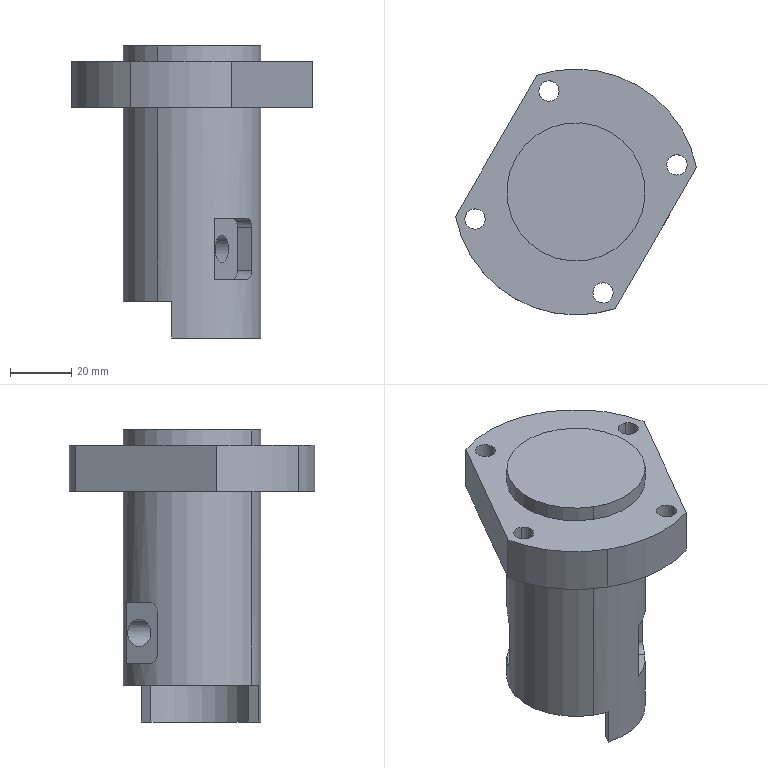Component | SolidWorks | SpindleFixtureAssemblyLeft-1_KLHFH009_38LocatingPin-1 | 1 solid | 86 faces | volume 154761 mm3 | cylinder 51 | plane 25 | cone 10 | commonest cylinder face diameters 8.8 x22 11 x8 6.6 x8 45 x4 6 x4 80 x3 38 x2 | material AISI Type A2 Tool Steel